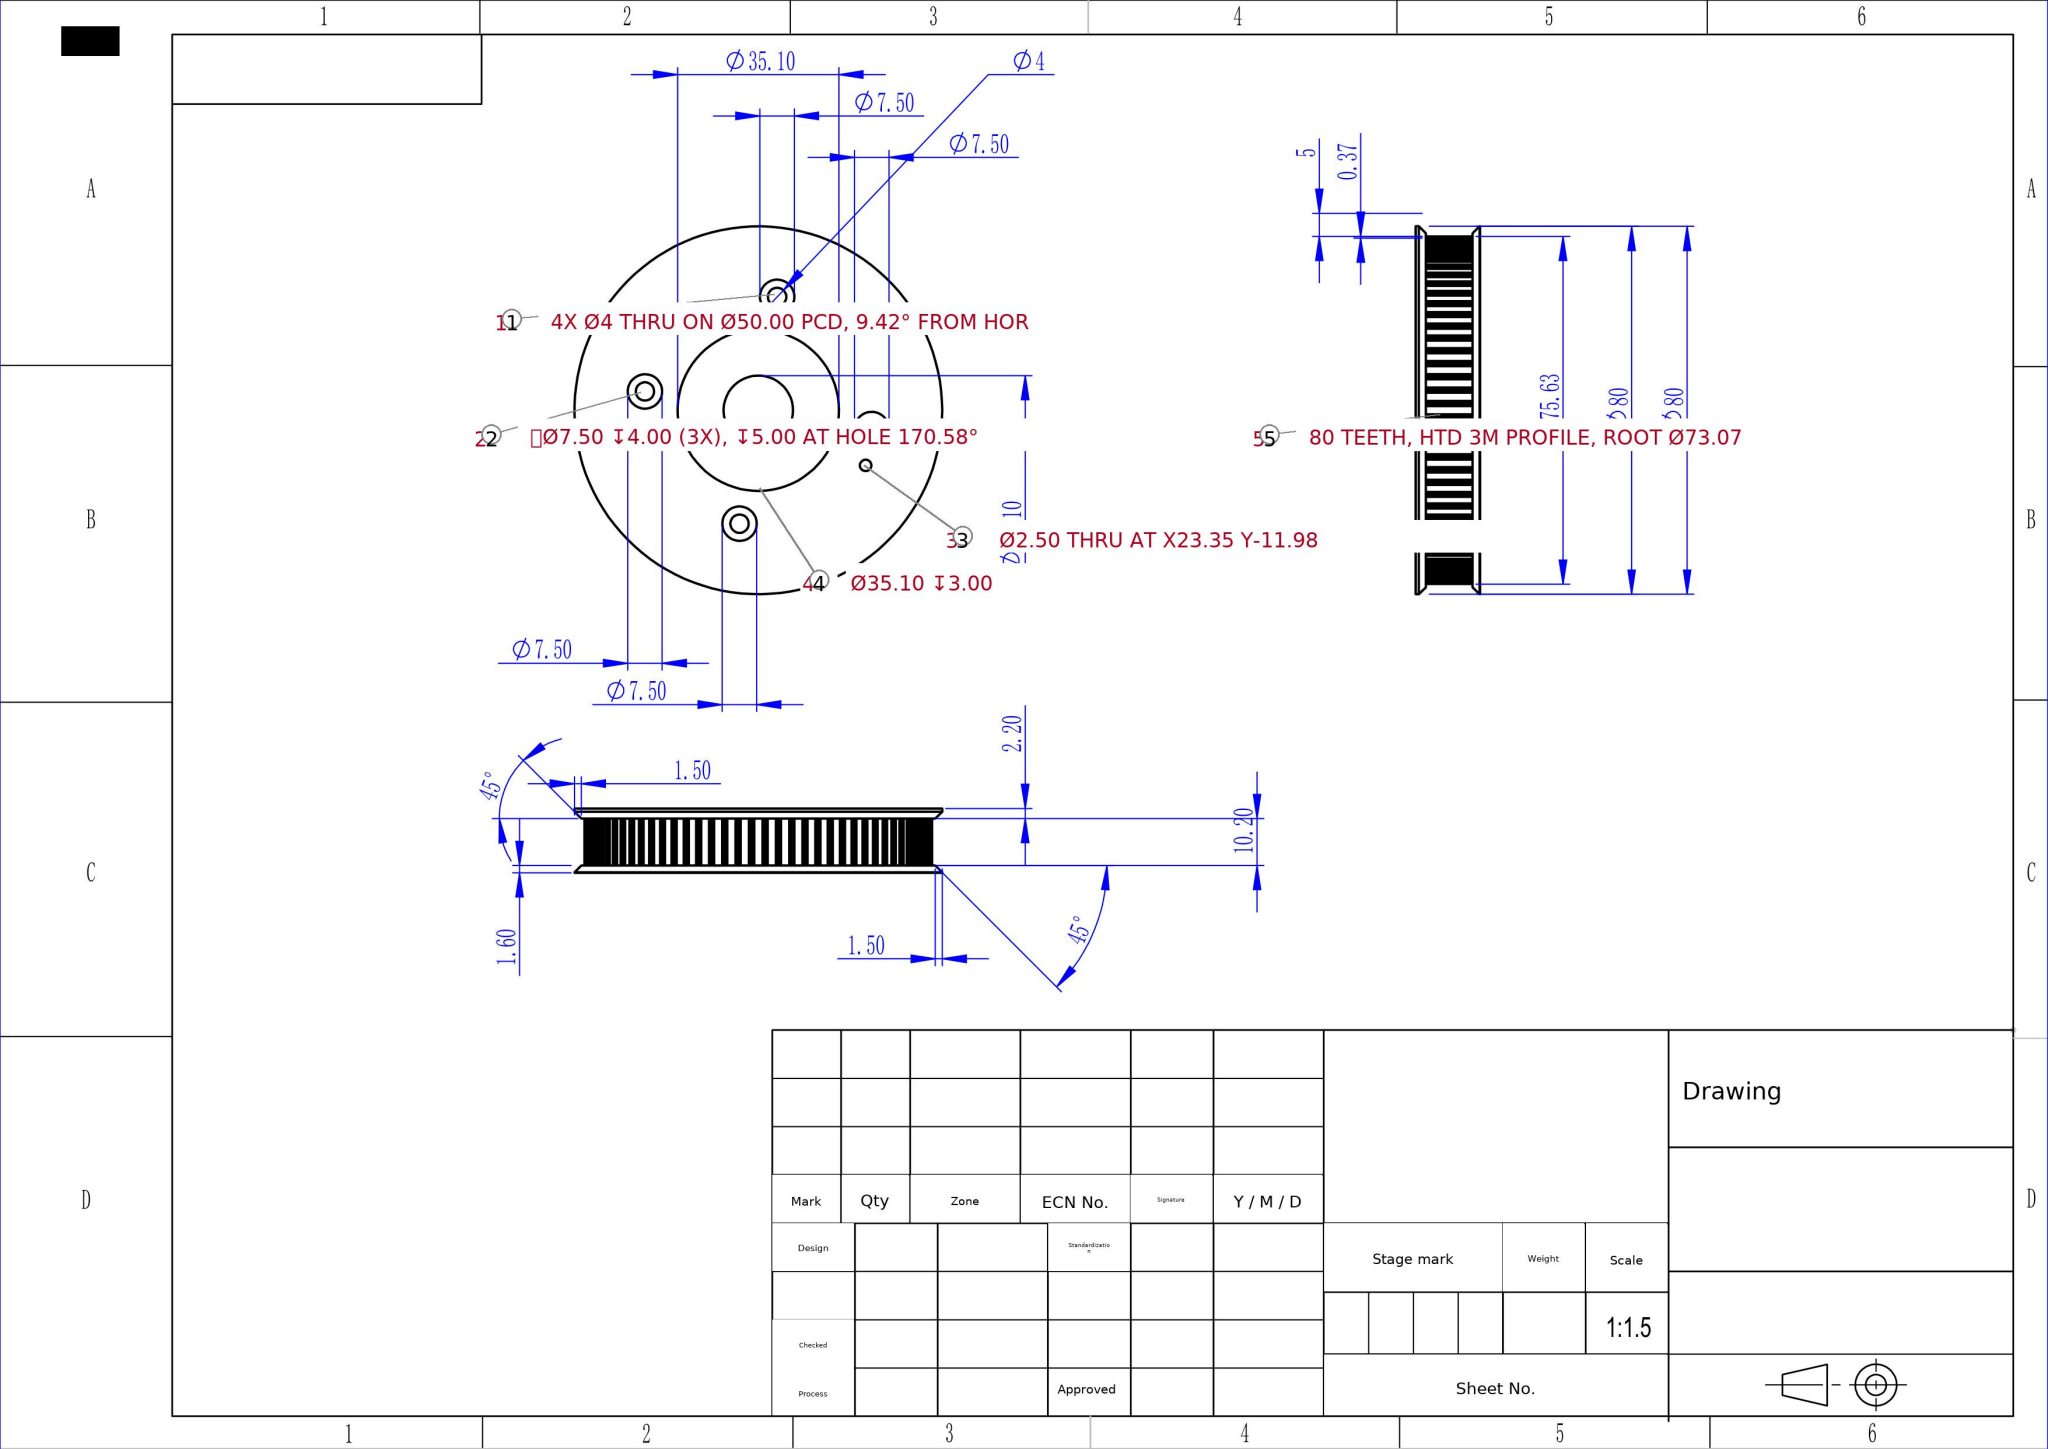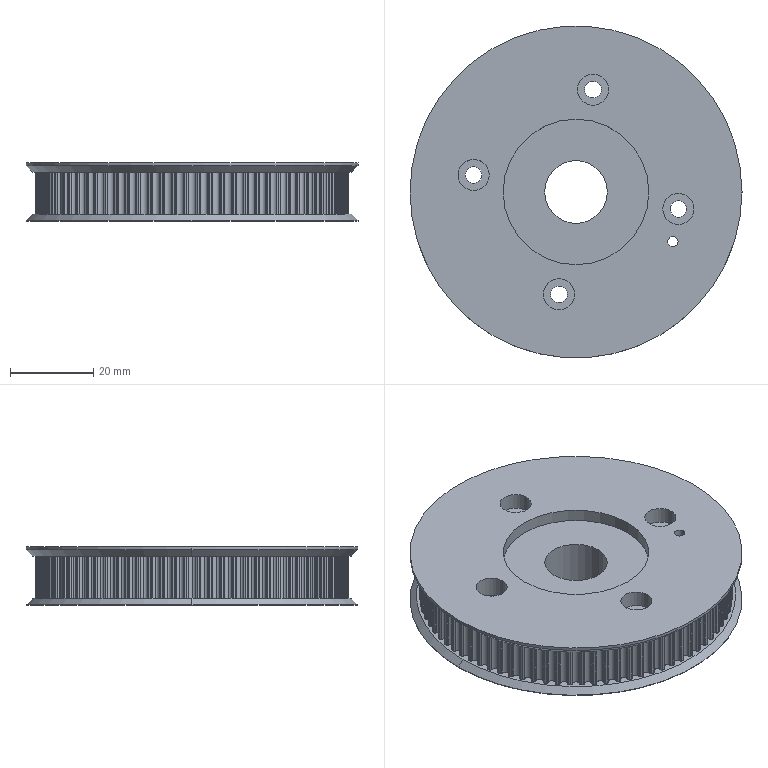Part | SolidWorks | mm | 1 solid | 594 faces | box 80 x 80 x 14 mm | volume 56534 mm3 | cylinder 421 | plane 169 | cone 4 | commonest cylinder face diameters 0.6 x198 1.82 x117 75.63 x80 7.5 x8 4 x8 80 x4 35.1 x2 2.5 x2